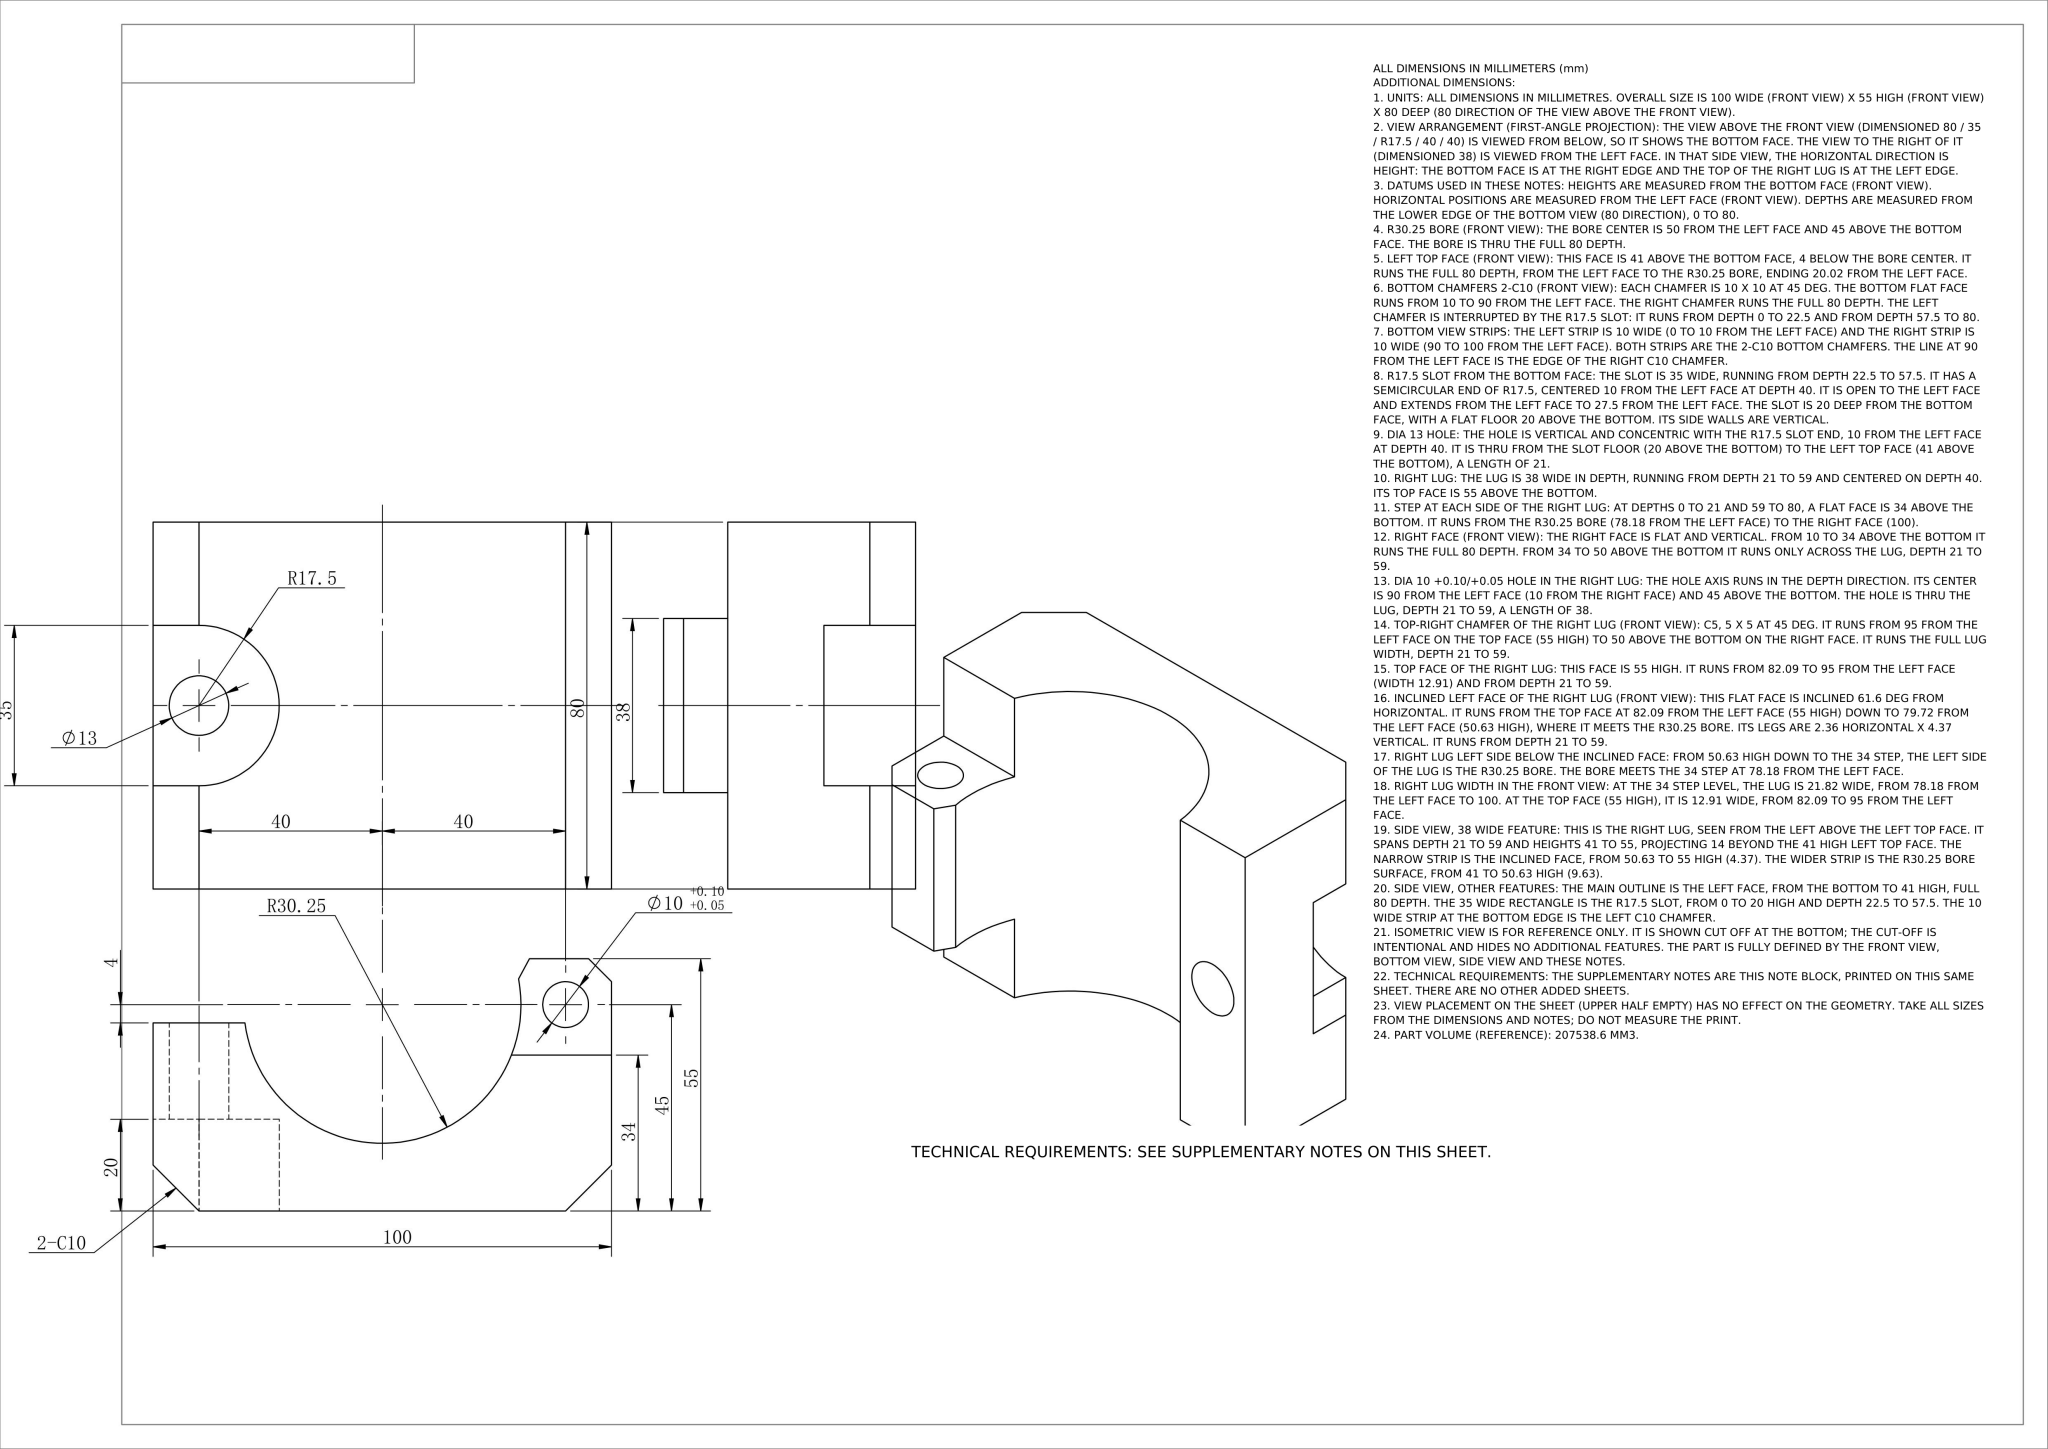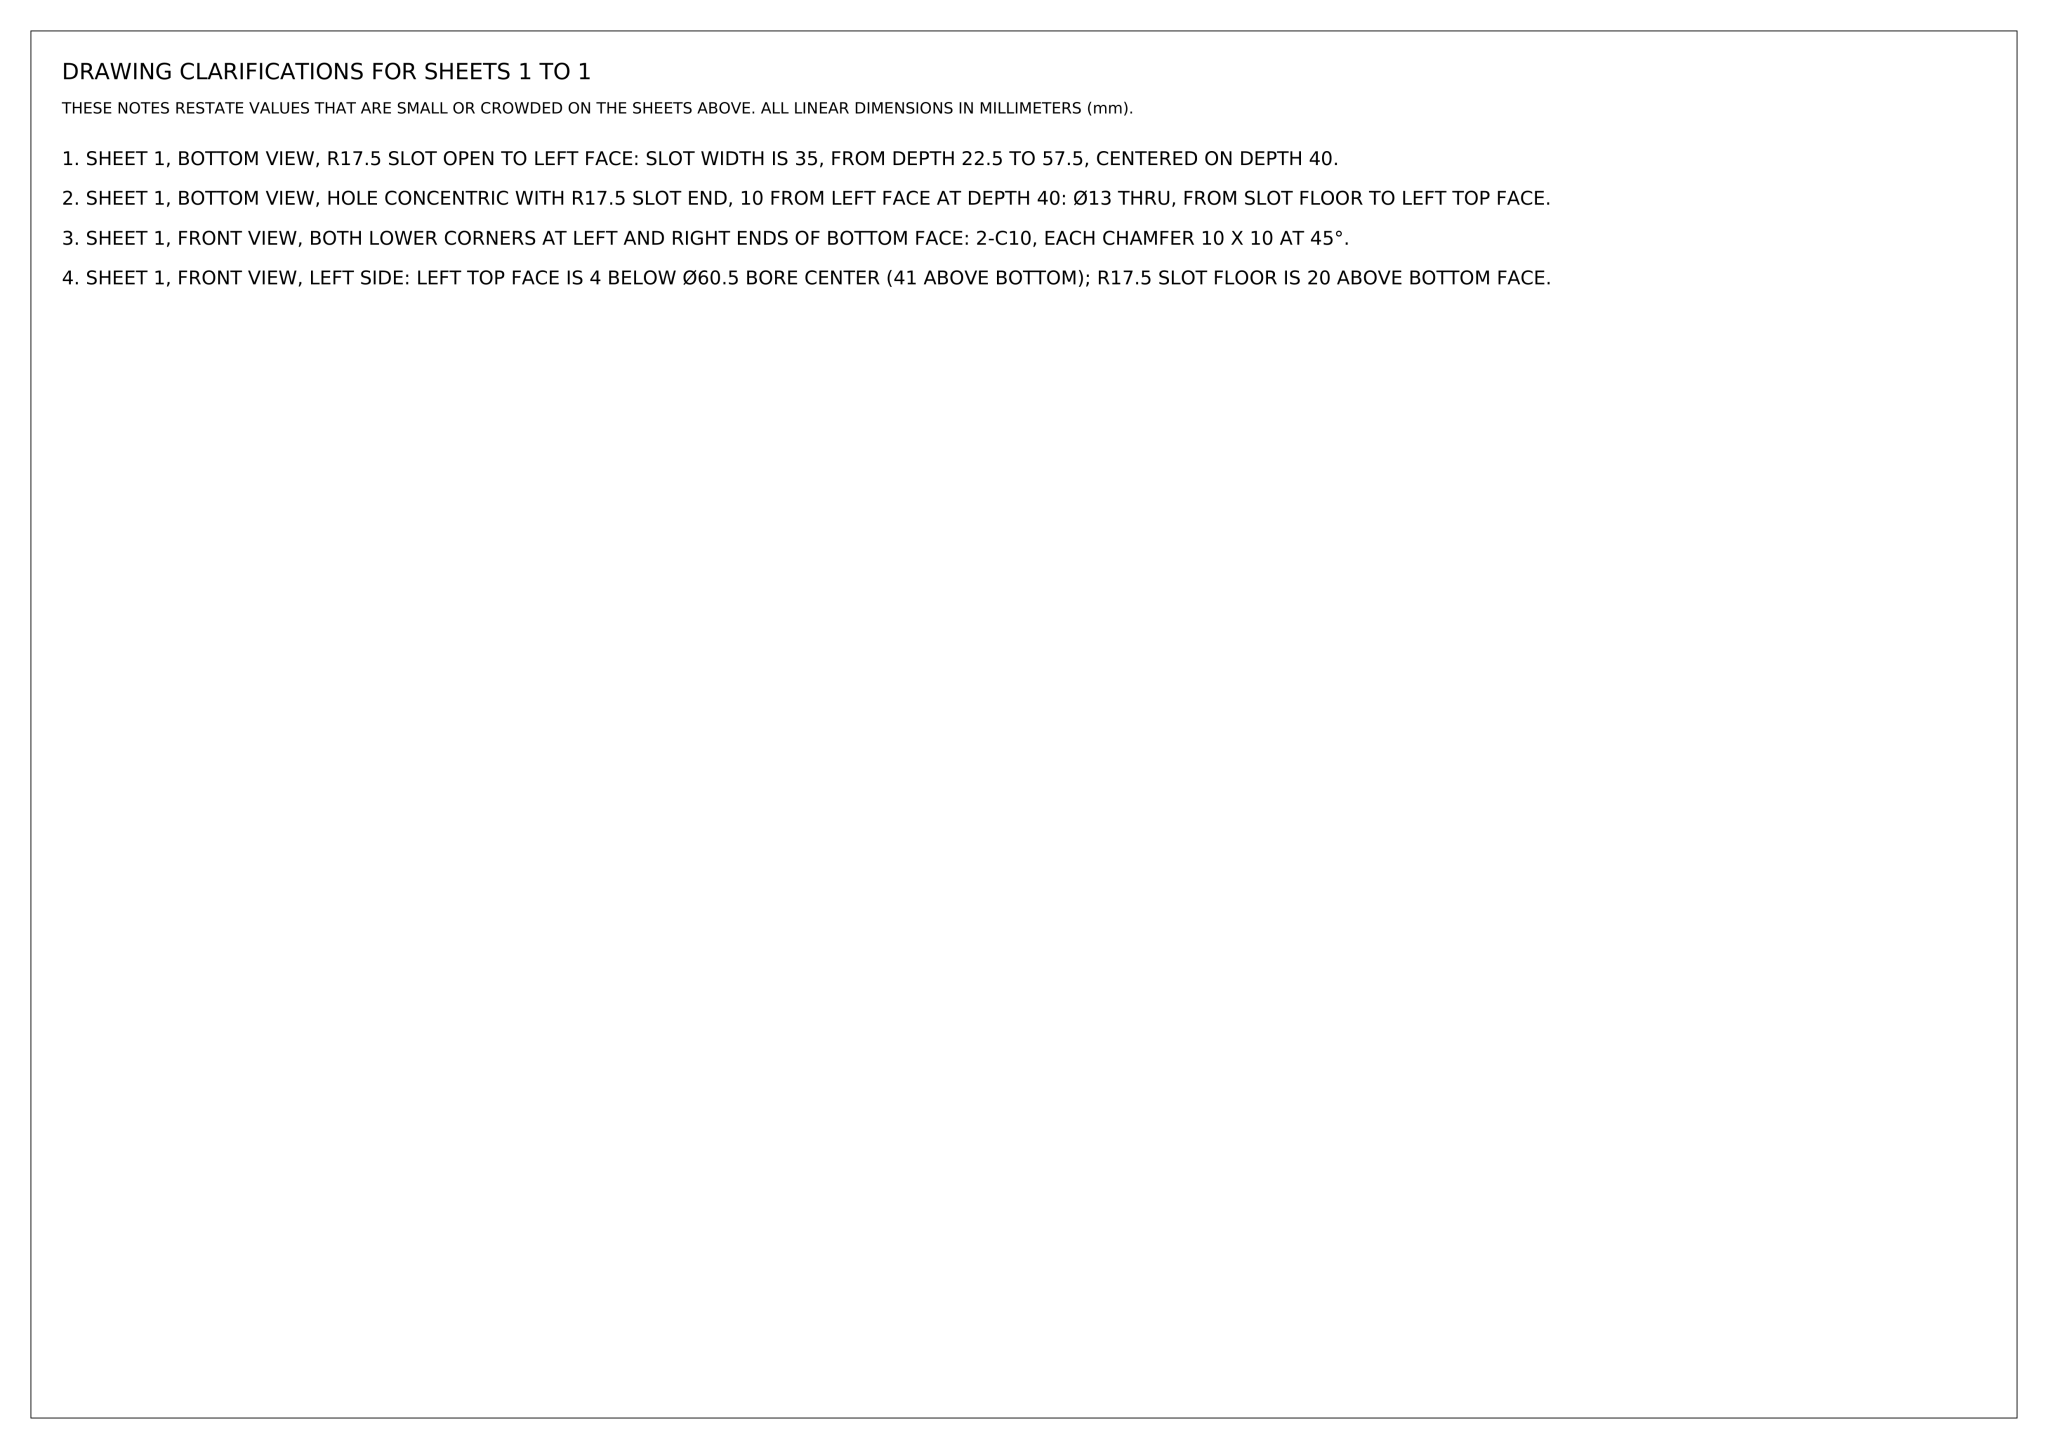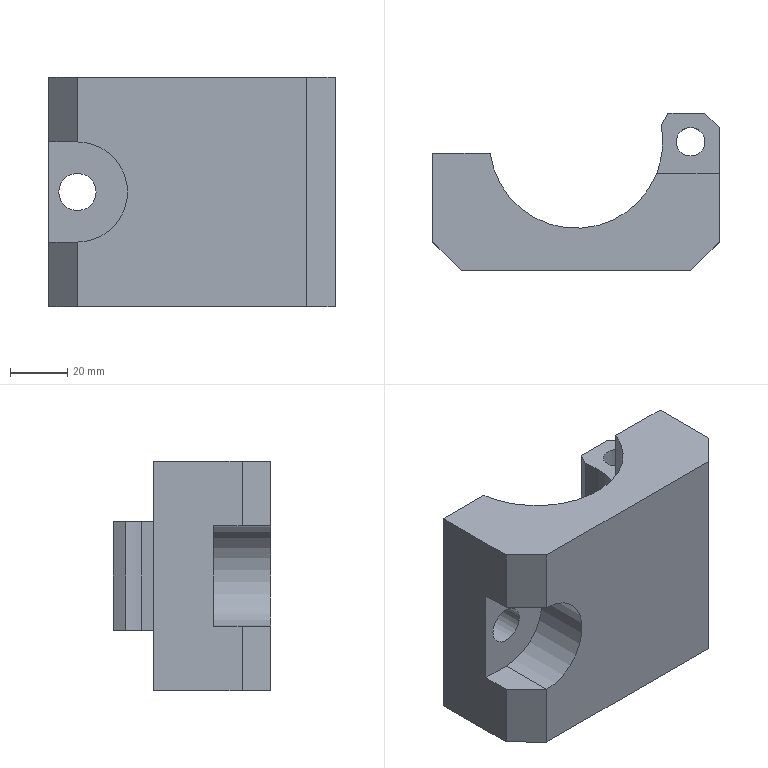Part | NX | mm | 1 solid | 26 faces | box 100 x 55 x 80 mm | volume 207539 mm3 | plane 19 | cylinder 7 | commonest cylinder face diameters 10 x2 60.5 x2 13 x2 35 x1
STEP:
#1=COLOUR_RGB('',0.502,0.502,1.);
#2=FILL_AREA_STYLE_COLOUR('',#1);
#3=FILL_AREA_STYLE('',(#2));
#4=SURFACE_STYLE_FILL_AREA(#3);
#5=SURFACE_SIDE_STYLE('',(#4));
#6=SURFACE_STYLE_USAGE(.BOTH.,#5);
#7=PRESENTATION_STYLE_ASSIGNMENT((#6));
#8=CARTESIAN_POINT('',(45.,-0.,21.));
#9=VERTEX_POINT('',#8);
#10=CARTESIAN_POINT('',(35.,-0.,21.));
#11=VERTEX_POINT('',#10);
#12=CARTESIAN_POINT('',(40.,-0.,21.));
#13=DIRECTION('',(0.,0.,-1.));
#14=DIRECTION('',(0.,-1.,0.));
#15=AXIS2_PLACEMENT_3D('',#12,#13,#14);
#16=CIRCLE('',#15,5.);
#17=EDGE_CURVE('',#9,#11,#16,.T.);
#18=ORIENTED_EDGE('',*,*,#17,.T.);
#19=CARTESIAN_POINT('',(35.,-0.,59.));
#20=VERTEX_POINT('',#19);
#21=CARTESIAN_POINT('',(35.,-0.,-199.));
#22=DIRECTION('',(-0.,-0.,1.));
#23=VECTOR('',#22,1000.);
#24=LINE('',#21,#23);
#25=EDGE_CURVE('',#11,#20,#24,.T.);
#26=ORIENTED_EDGE('',*,*,#25,.T.);
#27=CARTESIAN_POINT('',(45.,-0.,59.));
#28=VERTEX_POINT('',#27);
#29=CARTESIAN_POINT('',(40.,-0.,59.));
#30=DIRECTION('',(-0.,-0.,1.));
#31=DIRECTION('',(-1.,0.,0.));
#32=AXIS2_PLACEMENT_3D('',#29,#30,#31);
#33=CIRCLE('',#32,5.);
#34=EDGE_CURVE('',#20,#28,#33,.T.);
#35=ORIENTED_EDGE('',*,*,#34,.T.);
#36=CARTESIAN_POINT('',(45.,-0.,-199.));
#37=DIRECTION('',(-0.,-0.,1.));
#38=VECTOR('',#37,1000.);
#39=LINE('',#36,#38);
#40=EDGE_CURVE('',#9,#28,#39,.T.);
#41=ORIENTED_EDGE('',*,*,#40,.F.);
#42=EDGE_LOOP('',(#18,#26,#35,#41));
#43=FACE_OUTER_BOUND('',#42,.T.);
#44=CARTESIAN_POINT('',(40.,-0.,-199.));
#45=DIRECTION('',(-0.,-0.,1.));
#46=DIRECTION('',(1.,-0.,0.));
#47=AXIS2_PLACEMENT_3D('',#44,#45,#46);
#48=CYLINDRICAL_SURFACE('',#47,5.);
#49=ADVANCED_FACE('',(#43),#48,.F.);
#50=CARTESIAN_POINT('',(29.722,5.629,21.));
#51=VERTEX_POINT('',#50);
#52=CARTESIAN_POINT('',(30.25,-0.,21.));
#53=VERTEX_POINT('',#52);
#54=CARTESIAN_POINT('',(-0.,-0.,21.));
#55=DIRECTION('',(0.,0.,-1.));
#56=DIRECTION('',(-0.,-1.,-0.));
#57=AXIS2_PLACEMENT_3D('',#54,#55,#56);
#58=CIRCLE('',#57,30.25);
#59=EDGE_CURVE('',#51,#53,#58,.T.);
#60=ORIENTED_EDGE('',*,*,#59,.T.);
#61=CARTESIAN_POINT('',(30.25,-0.,59.));
#62=VERTEX_POINT('',#61);
#63=CARTESIAN_POINT('',(30.25,-0.,-199.));
#64=DIRECTION('',(-0.,-0.,1.));
#65=VECTOR('',#64,1000.);
#66=LINE('',#63,#65);
#67=EDGE_CURVE('',#53,#62,#66,.T.);
#68=ORIENTED_EDGE('',*,*,#67,.T.);
#69=CARTESIAN_POINT('',(29.722,5.629,59.));
#70=VERTEX_POINT('',#69);
#71=CARTESIAN_POINT('',(-0.,-0.,59.));
#72=DIRECTION('',(-0.,-0.,1.));
#73=DIRECTION('',(-1.,0.,0.));
#74=AXIS2_PLACEMENT_3D('',#71,#72,#73);
#75=CIRCLE('',#74,30.25);
#76=EDGE_CURVE('',#62,#70,#75,.T.);
#77=ORIENTED_EDGE('',*,*,#76,.T.);
#78=CARTESIAN_POINT('',(29.722,5.629,-199.));
#79=DIRECTION('',(0.,0.,-1.));
#80=VECTOR('',#79,1000.);
#81=LINE('',#78,#80);
#82=EDGE_CURVE('',#70,#51,#81,.T.);
#83=ORIENTED_EDGE('',*,*,#82,.T.);
#84=EDGE_LOOP('',(#60,#68,#77,#83));
#85=FACE_OUTER_BOUND('',#84,.T.);
#86=CARTESIAN_POINT('',(0.,0.,-199.));
#87=DIRECTION('',(-0.,-0.,1.));
#88=DIRECTION('',(1.,-0.,0.));
#89=AXIS2_PLACEMENT_3D('',#86,#87,#88);
#90=CYLINDRICAL_SURFACE('',#89,30.25);
#91=ADVANCED_FACE('',(#85),#90,.F.);
#92=CARTESIAN_POINT('',(-33.5,-25.,40.));
#93=VERTEX_POINT('',#92);
#94=CARTESIAN_POINT('',(-46.5,-25.,40.));
#95=VERTEX_POINT('',#94);
#96=CARTESIAN_POINT('',(-40.,-25.,40.));
#97=DIRECTION('',(-0.,1.,-0.));
#98=DIRECTION('',(0.,0.,-1.));
#99=AXIS2_PLACEMENT_3D('',#96,#97,#98);
#100=CIRCLE('',#99,6.5);
#101=EDGE_CURVE('',#93,#95,#100,.T.);
#102=ORIENTED_EDGE('',*,*,#101,.F.);
#103=CARTESIAN_POINT('',(-33.5,-4.,40.));
#104=VERTEX_POINT('',#103);
#105=CARTESIAN_POINT('',(-33.5,-75.,40.));
#106=DIRECTION('',(-0.,1.,-0.));
#107=VECTOR('',#106,1000.);
#108=LINE('',#105,#107);
#109=EDGE_CURVE('',#93,#104,#108,.T.);
#110=ORIENTED_EDGE('',*,*,#109,.T.);
#111=CARTESIAN_POINT('',(-46.5,-4.,40.));
#112=VERTEX_POINT('',#111);
#113=CARTESIAN_POINT('',(-40.,-4.,40.));
#114=DIRECTION('',(-0.,1.,-0.));
#115=DIRECTION('',(-1.,0.,0.));
#116=AXIS2_PLACEMENT_3D('',#113,#114,#115);
#117=CIRCLE('',#116,6.5);
#118=EDGE_CURVE('',#104,#112,#117,.T.);
#119=ORIENTED_EDGE('',*,*,#118,.T.);
#120=CARTESIAN_POINT('',(-46.5,-75.,40.));
#121=DIRECTION('',(-0.,1.,-0.));
#122=VECTOR('',#121,1000.);
#123=LINE('',#120,#122);
#124=EDGE_CURVE('',#95,#112,#123,.T.);
#125=ORIENTED_EDGE('',*,*,#124,.F.);
#126=EDGE_LOOP('',(#102,#110,#119,#125));
#127=FACE_OUTER_BOUND('',#126,.T.);
#128=CARTESIAN_POINT('',(-40.,-75.,40.));
#129=DIRECTION('',(-0.,1.,-0.));
#130=DIRECTION('',(-1.,0.,0.));
#131=AXIS2_PLACEMENT_3D('',#128,#129,#130);
#132=CYLINDRICAL_SURFACE('',#131,6.5);
#133=ADVANCED_FACE('',(#127),#132,.F.);
#134=CARTESIAN_POINT('',(-50.,-35.,57.5));
#135=VERTEX_POINT('',#134);
#136=CARTESIAN_POINT('',(-50.,-35.,80.));
#137=VERTEX_POINT('',#136);
#138=CARTESIAN_POINT('',(-50.,-35.,80.));
#139=DIRECTION('',(-0.,-0.,1.));
#140=VECTOR('',#139,1000.);
#141=LINE('',#138,#140);
#142=EDGE_CURVE('',#135,#137,#141,.T.);
#143=ORIENTED_EDGE('',*,*,#142,.F.);
#144=CARTESIAN_POINT('',(-40.,-45.,57.5));
#145=VERTEX_POINT('',#144);
#146=CARTESIAN_POINT('',(-40.,-45.,57.5));
#147=DIRECTION('',(0.7071,-0.7071,0.));
#148=VECTOR('',#147,1000.);
#149=LINE('',#146,#148);
#150=EDGE_CURVE('',#135,#145,#149,.T.);
#151=ORIENTED_EDGE('',*,*,#150,.T.);
#152=CARTESIAN_POINT('',(-40.,-45.,80.));
#153=VERTEX_POINT('',#152);
#154=CARTESIAN_POINT('',(-40.,-45.,80.));
#155=DIRECTION('',(0.,0.,-1.));
#156=VECTOR('',#155,1000.);
#157=LINE('',#154,#156);
#158=EDGE_CURVE('',#153,#145,#157,.T.);
#159=ORIENTED_EDGE('',*,*,#158,.F.);
#160=CARTESIAN_POINT('',(5.,-90.,80.));
#161=DIRECTION('',(0.7071,-0.7071,0.));
#162=VECTOR('',#161,1000.);
#163=LINE('',#160,#162);
#164=EDGE_CURVE('',#137,#153,#163,.T.);
#165=ORIENTED_EDGE('',*,*,#164,.F.);
#166=EDGE_LOOP('',(#143,#151,#159,#165));
#167=FACE_OUTER_BOUND('',#166,.T.);
#168=CARTESIAN_POINT('',(-40.,-45.,80.));
#169=DIRECTION('',(0.7071,0.7071,-0.));
#170=DIRECTION('',(-0.7071,0.7071,-0.));
#171=AXIS2_PLACEMENT_3D('',#168,#169,#170);
#172=PLANE('',#171);
#173=ADVANCED_FACE('',(#167),#172,.F.);
#174=CARTESIAN_POINT('',(-50.,-25.,57.5));
#175=VERTEX_POINT('',#174);
#176=CARTESIAN_POINT('',(-50.,45.,57.5));
#177=DIRECTION('',(-0.,1.,-0.));
#178=VECTOR('',#177,1000.);
#179=LINE('',#176,#178);
#180=EDGE_CURVE('',#135,#175,#179,.T.);
#181=ORIENTED_EDGE('',*,*,#180,.F.);
#182=ORIENTED_EDGE('',*,*,#142,.T.);
#183=CARTESIAN_POINT('',(-50.,-4.,80.));
#184=VERTEX_POINT('',#183);
#185=CARTESIAN_POINT('',(-50.,45.,80.));
#186=DIRECTION('',(0.,-1.,0.));
#187=VECTOR('',#186,1000.);
#188=LINE('',#185,#187);
#189=EDGE_CURVE('',#184,#137,#188,.T.);
#190=ORIENTED_EDGE('',*,*,#189,.F.);
#191=CARTESIAN_POINT('',(-50.,-4.,0.));
#192=VERTEX_POINT('',#191);
#193=CARTESIAN_POINT('',(-50.,-4.,-199.));
#194=DIRECTION('',(-0.,-0.,1.));
#195=VECTOR('',#194,1000.);
#196=LINE('',#193,#195);
#197=EDGE_CURVE('',#192,#184,#196,.T.);
#198=ORIENTED_EDGE('',*,*,#197,.F.);
#199=CARTESIAN_POINT('',(-50.,-35.,0.));
#200=VERTEX_POINT('',#199);
#201=CARTESIAN_POINT('',(-50.,45.,0.));
#202=DIRECTION('',(0.,-1.,0.));
#203=VECTOR('',#202,1000.);
#204=LINE('',#201,#203);
#205=EDGE_CURVE('',#192,#200,#204,.T.);
#206=ORIENTED_EDGE('',*,*,#205,.T.);
#207=CARTESIAN_POINT('',(-50.,-35.,22.5));
#208=VERTEX_POINT('',#207);
#209=CARTESIAN_POINT('',(-50.,-35.,80.));
#210=DIRECTION('',(-0.,-0.,1.));
#211=VECTOR('',#210,1000.);
#212=LINE('',#209,#211);
#213=EDGE_CURVE('',#200,#208,#212,.T.);
#214=ORIENTED_EDGE('',*,*,#213,.T.);
#215=CARTESIAN_POINT('',(-50.,-25.,22.5));
#216=VERTEX_POINT('',#215);
#217=CARTESIAN_POINT('',(-50.,45.,22.5));
#218=DIRECTION('',(0.,-1.,0.));
#219=VECTOR('',#218,1000.);
#220=LINE('',#217,#219);
#221=EDGE_CURVE('',#216,#208,#220,.T.);
#222=ORIENTED_EDGE('',*,*,#221,.F.);
#223=CARTESIAN_POINT('',(-50.,-25.,80.));
#224=DIRECTION('',(0.,0.,-1.));
#225=VECTOR('',#224,1000.);
#226=LINE('',#223,#225);
#227=EDGE_CURVE('',#175,#216,#226,.T.);
#228=ORIENTED_EDGE('',*,*,#227,.F.);
#229=EDGE_LOOP('',(#181,#182,#190,#198,#206,#214,#222,#228));
#230=FACE_OUTER_BOUND('',#229,.T.);
#231=CARTESIAN_POINT('',(-50.,45.,80.));
#232=DIRECTION('',(1.,0.,-0.));
#233=DIRECTION('',(-0.,1.,-0.));
#234=AXIS2_PLACEMENT_3D('',#231,#232,#233);
#235=PLANE('',#234);
#236=ADVANCED_FACE('',(#230),#235,.F.);
#237=CARTESIAN_POINT('',(-40.,-45.,22.5));
#238=VERTEX_POINT('',#237);
#239=CARTESIAN_POINT('',(-40.,-45.,0.));
#240=VERTEX_POINT('',#239);
#241=CARTESIAN_POINT('',(-40.,-45.,80.));
#242=DIRECTION('',(0.,0.,-1.));
#243=VECTOR('',#242,1000.);
#244=LINE('',#241,#243);
#245=EDGE_CURVE('',#238,#240,#244,.T.);
#246=ORIENTED_EDGE('',*,*,#245,.F.);
#247=CARTESIAN_POINT('',(-40.,-45.,22.5));
#248=DIRECTION('',(-0.7071,0.7071,0.));
#249=VECTOR('',#248,1000.);
#250=LINE('',#247,#249);
#251=EDGE_CURVE('',#238,#208,#250,.T.);
#252=ORIENTED_EDGE('',*,*,#251,.T.);
#253=ORIENTED_EDGE('',*,*,#213,.F.);
#254=CARTESIAN_POINT('',(-40.,-45.,0.));
#255=DIRECTION('',(-0.7071,0.7071,-0.));
#256=VECTOR('',#255,1000.);
#257=LINE('',#254,#256);
#258=EDGE_CURVE('',#240,#200,#257,.T.);
#259=ORIENTED_EDGE('',*,*,#258,.F.);
#260=EDGE_LOOP('',(#246,#252,#253,#259));
#261=FACE_OUTER_BOUND('',#260,.T.);
#262=CARTESIAN_POINT('',(-40.,-45.,80.));
#263=DIRECTION('',(0.7071,0.7071,-0.));
#264=DIRECTION('',(-0.7071,0.7071,-0.));
#265=AXIS2_PLACEMENT_3D('',#262,#263,#264);
#266=PLANE('',#265);
#267=ADVANCED_FACE('',(#261),#266,.F.);
#268=CARTESIAN_POINT('',(-40.,-45.,40.));
#269=DIRECTION('',(0.,-1.,0.));
#270=DIRECTION('',(0.,0.,-1.));
#271=AXIS2_PLACEMENT_3D('',#268,#269,#270);
#272=CIRCLE('',#271,17.5);
#273=EDGE_CURVE('',#238,#145,#272,.T.);
#274=ORIENTED_EDGE('',*,*,#273,.T.);
#275=CARTESIAN_POINT('',(-40.,-25.,57.5));
#276=VERTEX_POINT('',#275);
#277=CARTESIAN_POINT('',(-40.,-65.,57.5));
#278=DIRECTION('',(-0.,1.,-0.));
#279=VECTOR('',#278,1000.);
#280=LINE('',#277,#279);
#281=EDGE_CURVE('',#145,#276,#280,.T.);
#282=ORIENTED_EDGE('',*,*,#281,.T.);
#283=CARTESIAN_POINT('',(-40.,-25.,22.5));
#284=VERTEX_POINT('',#283);
#285=CARTESIAN_POINT('',(-40.,-25.,40.));
#286=DIRECTION('',(0.,-1.,0.));
#287=DIRECTION('',(0.,0.,-1.));
#288=AXIS2_PLACEMENT_3D('',#285,#286,#287);
#289=CIRCLE('',#288,17.5);
#290=EDGE_CURVE('',#284,#276,#289,.T.);
#291=ORIENTED_EDGE('',*,*,#290,.F.);
#292=CARTESIAN_POINT('',(-40.,-65.,22.5));
#293=DIRECTION('',(-0.,1.,-0.));
#294=VECTOR('',#293,1000.);
#295=LINE('',#292,#294);
#296=EDGE_CURVE('',#238,#284,#295,.T.);
#297=ORIENTED_EDGE('',*,*,#296,.F.);
#298=EDGE_LOOP('',(#274,#282,#291,#297));
#299=FACE_OUTER_BOUND('',#298,.T.);
#300=CARTESIAN_POINT('',(-40.,-25.,40.));
#301=DIRECTION('',(0.,-1.,0.));
#302=DIRECTION('',(0.,0.,-1.));
#303=AXIS2_PLACEMENT_3D('',#300,#301,#302);
#304=CYLINDRICAL_SURFACE('',#303,17.5);
#305=ADVANCED_FACE('',(#299),#304,.F.);
#306=ORIENTED_EDGE('',*,*,#109,.F.);
#307=CARTESIAN_POINT('',(-40.,-25.,40.));
#308=DIRECTION('',(-0.,1.,-0.));
#309=DIRECTION('',(0.,0.,-1.));
#310=AXIS2_PLACEMENT_3D('',#307,#308,#309);
#311=CIRCLE('',#310,6.5);
#312=EDGE_CURVE('',#95,#93,#311,.T.);
#313=ORIENTED_EDGE('',*,*,#312,.F.);
#314=ORIENTED_EDGE('',*,*,#124,.T.);
#315=CARTESIAN_POINT('',(-40.,-4.,40.));
#316=DIRECTION('',(-0.,1.,-0.));
#317=DIRECTION('',(-1.,0.,0.));
#318=AXIS2_PLACEMENT_3D('',#315,#316,#317);
#319=CIRCLE('',#318,6.5);
#320=EDGE_CURVE('',#112,#104,#319,.T.);
#321=ORIENTED_EDGE('',*,*,#320,.T.);
#322=EDGE_LOOP('',(#306,#313,#314,#321));
#323=FACE_OUTER_BOUND('',#322,.T.);
#324=CARTESIAN_POINT('',(-40.,-75.,40.));
#325=DIRECTION('',(-0.,1.,-0.));
#326=DIRECTION('',(-1.,0.,0.));
#327=AXIS2_PLACEMENT_3D('',#324,#325,#326);
#328=CYLINDRICAL_SURFACE('',#327,6.5);
#329=ADVANCED_FACE('',(#323),#328,.F.);
#330=CARTESIAN_POINT('',(50.,-35.,80.));
#331=VERTEX_POINT('',#330);
#332=CARTESIAN_POINT('',(50.,-11.,80.));
#333=VERTEX_POINT('',#332);
#334=CARTESIAN_POINT('',(50.,45.,80.));
#335=DIRECTION('',(-0.,1.,-0.));
#336=VECTOR('',#335,1000.);
#337=LINE('',#334,#336);
#338=EDGE_CURVE('',#331,#333,#337,.T.);
#339=ORIENTED_EDGE('',*,*,#338,.F.);
#340=CARTESIAN_POINT('',(50.,-35.,0.));
#341=VERTEX_POINT('',#340);
#342=CARTESIAN_POINT('',(50.,-35.,80.));
#343=DIRECTION('',(0.,0.,-1.));
#344=VECTOR('',#343,1000.);
#345=LINE('',#342,#344);
#346=EDGE_CURVE('',#331,#341,#345,.T.);
#347=ORIENTED_EDGE('',*,*,#346,.T.);
#348=CARTESIAN_POINT('',(50.,-11.,0.));
#349=VERTEX_POINT('',#348);
#350=CARTESIAN_POINT('',(50.,45.,0.));
#351=DIRECTION('',(-0.,1.,-0.));
#352=VECTOR('',#351,1000.);
#353=LINE('',#350,#352);
#354=EDGE_CURVE('',#341,#349,#353,.T.);
#355=ORIENTED_EDGE('',*,*,#354,.T.);
#356=CARTESIAN_POINT('',(50.,-11.,21.));
#357=VERTEX_POINT('',#356);
#358=CARTESIAN_POINT('',(50.,-11.,0.));
#359=DIRECTION('',(0.,0.,-1.));
#360=VECTOR('',#359,1000.);
#361=LINE('',#358,#360);
#362=EDGE_CURVE('',#357,#349,#361,.T.);
#363=ORIENTED_EDGE('',*,*,#362,.F.);
#364=CARTESIAN_POINT('',(50.,5.,21.));
#365=VERTEX_POINT('',#364);
#366=CARTESIAN_POINT('',(50.,10.,21.));
#367=DIRECTION('',(0.,-1.,-0.));
#368=VECTOR('',#367,1000.);
#369=LINE('',#366,#368);
#370=EDGE_CURVE('',#365,#357,#369,.T.);
#371=ORIENTED_EDGE('',*,*,#370,.F.);
#372=CARTESIAN_POINT('',(50.,5.,59.));
#373=VERTEX_POINT('',#372);
#374=CARTESIAN_POINT('',(50.,5.,80.));
#375=DIRECTION('',(-0.,-0.,1.));
#376=VECTOR('',#375,1000.);
#377=LINE('',#374,#376);
#378=EDGE_CURVE('',#365,#373,#377,.T.);
#379=ORIENTED_EDGE('',*,*,#378,.T.);
#380=CARTESIAN_POINT('',(50.,-11.,59.));
#381=VERTEX_POINT('',#380);
#382=CARTESIAN_POINT('',(50.,10.,59.));
#383=DIRECTION('',(-0.,1.,-0.));
#384=VECTOR('',#383,1000.);
#385=LINE('',#382,#384);
#386=EDGE_CURVE('',#381,#373,#385,.T.);
#387=ORIENTED_EDGE('',*,*,#386,.F.);
#388=CARTESIAN_POINT('',(50.,-11.,80.));
#389=DIRECTION('',(0.,0.,-1.));
#390=VECTOR('',#389,1000.);
#391=LINE('',#388,#390);
#392=EDGE_CURVE('',#333,#381,#391,.T.);
#393=ORIENTED_EDGE('',*,*,#392,.F.);
#394=EDGE_LOOP('',(#339,#347,#355,#363,#371,#379,#387,#393));
#395=FACE_OUTER_BOUND('',#394,.T.);
#396=CARTESIAN_POINT('',(50.,45.,80.));
#397=DIRECTION('',(-1.,-0.,0.));
#398=DIRECTION('',(0.,-1.,0.));
#399=AXIS2_PLACEMENT_3D('',#396,#397,#398);
#400=PLANE('',#399);
#401=ADVANCED_FACE('',(#395),#400,.F.);
#402=ORIENTED_EDGE('',*,*,#158,.T.);
#403=ORIENTED_EDGE('',*,*,#273,.F.);
#404=ORIENTED_EDGE('',*,*,#245,.T.);
#405=CARTESIAN_POINT('',(40.,-45.,0.));
#406=VERTEX_POINT('',#405);
#407=CARTESIAN_POINT('',(-50.,-45.,0.));
#408=DIRECTION('',(1.,-0.,-0.));
#409=VECTOR('',#408,1000.);
#410=LINE('',#407,#409);
#411=EDGE_CURVE('',#240,#406,#410,.T.);
#412=ORIENTED_EDGE('',*,*,#411,.T.);
#413=CARTESIAN_POINT('',(40.,-45.,80.));
#414=VERTEX_POINT('',#413);
#415=CARTESIAN_POINT('',(40.,-45.,80.));
#416=DIRECTION('',(-0.,-0.,1.));
#417=VECTOR('',#416,1000.);
#418=LINE('',#415,#417);
#419=EDGE_CURVE('',#406,#414,#418,.T.);
#420=ORIENTED_EDGE('',*,*,#419,.T.);
#421=CARTESIAN_POINT('',(-50.,-45.,80.));
#422=DIRECTION('',(1.,-0.,-0.));
#423=VECTOR('',#422,1000.);
#424=LINE('',#421,#423);
#425=EDGE_CURVE('',#153,#414,#424,.T.);
#426=ORIENTED_EDGE('',*,*,#425,.F.);
#427=EDGE_LOOP('',(#402,#403,#404,#412,#420,#426));
#428=FACE_OUTER_BOUND('',#427,.T.);
#429=CARTESIAN_POINT('',(-50.,-45.,80.));
#430=DIRECTION('',(-0.,1.,0.));
#431=DIRECTION('',(-0.,-0.,1.));
#432=AXIS2_PLACEMENT_3D('',#429,#430,#431);
#433=PLANE('',#432);
#434=ADVANCED_FACE('',(#428),#433,.F.);
#435=ORIENTED_EDGE('',*,*,#189,.T.);
#436=ORIENTED_EDGE('',*,*,#164,.T.);
#437=ORIENTED_EDGE('',*,*,#425,.T.);
#438=CARTESIAN_POINT('',(45.,-40.,80.));
#439=DIRECTION('',(0.7071,0.7071,-0.));
#440=VECTOR('',#439,1000.);
#441=LINE('',#438,#440);
#442=EDGE_CURVE('',#414,#331,#441,.T.);
#443=ORIENTED_EDGE('',*,*,#442,.T.);
#444=ORIENTED_EDGE('',*,*,#338,.T.);
#445=CARTESIAN_POINT('',(28.179,-11.,80.));
#446=VERTEX_POINT('',#445);
#447=CARTESIAN_POINT('',(-9.,-11.,80.));
#448=DIRECTION('',(1.,-0.,-0.));
#449=VECTOR('',#448,1000.);
#450=LINE('',#447,#449);
#451=EDGE_CURVE('',#446,#333,#450,.T.);
#452=ORIENTED_EDGE('',*,*,#451,.F.);
#453=CARTESIAN_POINT('',(-29.984,-4.,80.));
#454=VERTEX_POINT('',#453);
#455=CARTESIAN_POINT('',(-0.,-0.,80.));
#456=DIRECTION('',(-0.,-0.,1.));
#457=DIRECTION('',(1.,-0.,0.));
#458=AXIS2_PLACEMENT_3D('',#455,#456,#457);
#459=CIRCLE('',#458,30.25);
#460=EDGE_CURVE('',#454,#446,#459,.T.);
#461=ORIENTED_EDGE('',*,*,#460,.F.);
#462=CARTESIAN_POINT('',(0.,-4.,80.));
#463=DIRECTION('',(1.,-0.,-0.));
#464=VECTOR('',#463,1000.);
#465=LINE('',#462,#464);
#466=EDGE_CURVE('',#184,#454,#465,.T.);
#467=ORIENTED_EDGE('',*,*,#466,.F.);
#468=EDGE_LOOP('',(#435,#436,#437,#443,#444,#452,#461,#467));
#469=FACE_OUTER_BOUND('',#468,.T.);
#470=CARTESIAN_POINT('',(50.,-45.,80.));
#471=DIRECTION('',(0.,-0.,1.));
#472=DIRECTION('',(1.,-0.,-0.));
#473=AXIS2_PLACEMENT_3D('',#470,#471,#472);
#474=PLANE('',#473);
#475=ADVANCED_FACE('',(#469),#474,.T.);
#476=ORIENTED_EDGE('',*,*,#411,.F.);
#477=ORIENTED_EDGE('',*,*,#258,.T.);
#478=ORIENTED_EDGE('',*,*,#205,.F.);
#479=CARTESIAN_POINT('',(-29.984,-4.,0.));
#480=VERTEX_POINT('',#479);
#481=CARTESIAN_POINT('',(50.,-4.,0.));
#482=DIRECTION('',(1.,-0.,-0.));
#483=VECTOR('',#482,1000.);
#484=LINE('',#481,#483);
#485=EDGE_CURVE('',#192,#480,#484,.T.);
#486=ORIENTED_EDGE('',*,*,#485,.T.);
#487=CARTESIAN_POINT('',(28.179,-11.,0.));
#488=VERTEX_POINT('',#487);
#489=CARTESIAN_POINT('',(0.,0.,0.));
#490=DIRECTION('',(-0.,-0.,1.));
#491=DIRECTION('',(1.,-0.,-0.));
#492=AXIS2_PLACEMENT_3D('',#489,#490,#491);
#493=CIRCLE('',#492,30.25);
#494=EDGE_CURVE('',#480,#488,#493,.T.);
#495=ORIENTED_EDGE('',*,*,#494,.T.);
#496=CARTESIAN_POINT('',(-9.,-11.,0.));
#497=DIRECTION('',(1.,-0.,-0.));
#498=VECTOR('',#497,1000.);
#499=LINE('',#496,#498);
#500=EDGE_CURVE('',#488,#349,#499,.T.);
#501=ORIENTED_EDGE('',*,*,#500,.T.);
#502=ORIENTED_EDGE('',*,*,#354,.F.);
#503=CARTESIAN_POINT('',(50.,-35.,0.));
#504=DIRECTION('',(-0.7071,-0.7071,0.));
#505=VECTOR('',#504,1000.);
#506=LINE('',#503,#505);
#507=EDGE_CURVE('',#341,#406,#506,.T.);
#508=ORIENTED_EDGE('',*,*,#507,.T.);
#509=EDGE_LOOP('',(#476,#477,#478,#486,#495,#501,#502,#508));
#510=FACE_OUTER_BOUND('',#509,.T.);
#511=CARTESIAN_POINT('',(50.,-45.,0.));
#512=DIRECTION('',(0.,-0.,1.));
#513=DIRECTION('',(1.,-0.,-0.));
#514=AXIS2_PLACEMENT_3D('',#511,#512,#513);
#515=PLANE('',#514);
#516=ADVANCED_FACE('',(#510),#515,.F.);
#517=ORIENTED_EDGE('',*,*,#67,.F.);
#518=CARTESIAN_POINT('',(28.179,-11.,21.));
#519=VERTEX_POINT('',#518);
#520=CARTESIAN_POINT('',(-0.,-0.,21.));
#521=DIRECTION('',(0.,0.,-1.));
#522=DIRECTION('',(0.,-1.,-0.));
#523=AXIS2_PLACEMENT_3D('',#520,#521,#522);
#524=CIRCLE('',#523,30.25);
#525=EDGE_CURVE('',#53,#519,#524,.T.);
#526=ORIENTED_EDGE('',*,*,#525,.T.);
#527=CARTESIAN_POINT('',(28.179,-11.,-199.));
#528=DIRECTION('',(0.,0.,-1.));
#529=VECTOR('',#528,1000.);
#530=LINE('',#527,#529);
#531=EDGE_CURVE('',#519,#488,#530,.T.);
#532=ORIENTED_EDGE('',*,*,#531,.T.);
#533=ORIENTED_EDGE('',*,*,#494,.F.);
#534=CARTESIAN_POINT('',(-29.984,-4.,-199.));
#535=DIRECTION('',(-0.,-0.,1.));
#536=VECTOR('',#535,1000.);
#537=LINE('',#534,#536);
#538=EDGE_CURVE('',#480,#454,#537,.T.);
#539=ORIENTED_EDGE('',*,*,#538,.T.);
#540=ORIENTED_EDGE('',*,*,#460,.T.);
#541=CARTESIAN_POINT('',(28.179,-11.,59.));
#542=VERTEX_POINT('',#541);
#543=CARTESIAN_POINT('',(28.179,-11.,-199.));
#544=DIRECTION('',(0.,0.,-1.));
#545=VECTOR('',#544,1000.);
#546=LINE('',#543,#545);
#547=EDGE_CURVE('',#446,#542,#546,.T.);
#548=ORIENTED_EDGE('',*,*,#547,.T.);
#549=CARTESIAN_POINT('',(-0.,-0.,59.));
#550=DIRECTION('',(-0.,-0.,1.));
#551=DIRECTION('',(-1.,0.,0.));
#552=AXIS2_PLACEMENT_3D('',#549,#550,#551);
#553=CIRCLE('',#552,30.25);
#554=EDGE_CURVE('',#542,#62,#553,.T.);
#555=ORIENTED_EDGE('',*,*,#554,.T.);
#556=EDGE_LOOP('',(#517,#526,#532,#533,#539,#540,#548,#555));
#557=FACE_OUTER_BOUND('',#556,.T.);
#558=CARTESIAN_POINT('',(0.,0.,-199.));
#559=DIRECTION('',(-0.,-0.,1.));
#560=DIRECTION('',(1.,-0.,0.));
#561=AXIS2_PLACEMENT_3D('',#558,#559,#560);
#562=CYLINDRICAL_SURFACE('',#561,30.25);
#563=ADVANCED_FACE('',(#557),#562,.F.);
#564=ORIENTED_EDGE('',*,*,#25,.F.);
#565=CARTESIAN_POINT('',(40.,-0.,21.));
#566=DIRECTION('',(0.,0.,-1.));
#567=DIRECTION('',(0.,-1.,0.));
#568=AXIS2_PLACEMENT_3D('',#565,#566,#567);
#569=CIRCLE('',#568,5.);
#570=EDGE_CURVE('',#11,#9,#569,.T.);
#571=ORIENTED_EDGE('',*,*,#570,.T.);
#572=ORIENTED_EDGE('',*,*,#40,.T.);
#573=CARTESIAN_POINT('',(40.,-0.,59.));
#574=DIRECTION('',(-0.,-0.,1.));
#575=DIRECTION('',(-1.,0.,0.));
#576=AXIS2_PLACEMENT_3D('',#573,#574,#575);
#577=CIRCLE('',#576,5.);
#578=EDGE_CURVE('',#28,#20,#577,.T.);
#579=ORIENTED_EDGE('',*,*,#578,.T.);
#580=EDGE_LOOP('',(#564,#571,#572,#579));
#581=FACE_OUTER_BOUND('',#580,.T.);
#582=CARTESIAN_POINT('',(40.,-0.,-199.));
#583=DIRECTION('',(-0.,-0.,1.));
#584=DIRECTION('',(1.,-0.,0.));
#585=AXIS2_PLACEMENT_3D('',#582,#583,#584);
#586=CYLINDRICAL_SURFACE('',#585,5.);
#587=ADVANCED_FACE('',(#581),#586,.F.);
#588=CARTESIAN_POINT('',(45.,10.,59.));
#589=VERTEX_POINT('',#588);
#590=CARTESIAN_POINT('',(45.,10.,21.));
#591=VERTEX_POINT('',#590);
#592=CARTESIAN_POINT('',(45.,10.,-199.));
#593=DIRECTION('',(0.,0.,-1.));
#594=VECTOR('',#593,1000.);
#595=LINE('',#592,#594);
#596=EDGE_CURVE('',#589,#591,#595,.T.);
#597=ORIENTED_EDGE('',*,*,#596,.T.);
#598=CARTESIAN_POINT('',(32.086,10.,21.));
#599=VERTEX_POINT('',#598);
#600=CARTESIAN_POINT('',(-9.,10.,21.));
#601=DIRECTION('',(1.,-0.,-0.));
#602=VECTOR('',#601,1000.);
#603=LINE('',#600,#602);
#604=EDGE_CURVE('',#599,#591,#603,.T.);
#605=ORIENTED_EDGE('',*,*,#604,.F.);
#606=CARTESIAN_POINT('',(32.086,10.,59.));
#607=VERTEX_POINT('',#606);
#608=CARTESIAN_POINT('',(32.086,10.,-199.));
#609=DIRECTION('',(-0.,-0.,1.));
#610=VECTOR('',#609,1000.);
#611=LINE('',#608,#610);
#612=EDGE_CURVE('',#599,#607,#611,.T.);
#613=ORIENTED_EDGE('',*,*,#612,.T.);
#614=CARTESIAN_POINT('',(-9.,10.,59.));
#615=DIRECTION('',(1.,-0.,-0.));
#616=VECTOR('',#615,1000.);
#617=LINE('',#614,#616);
#618=EDGE_CURVE('',#607,#589,#617,.T.);
#619=ORIENTED_EDGE('',*,*,#618,.T.);
#620=EDGE_LOOP('',(#597,#605,#613,#619));
#621=FACE_OUTER_BOUND('',#620,.T.);
#622=CARTESIAN_POINT('',(50.,10.,-199.));
#623=DIRECTION('',(-0.,-1.,0.));
#624=DIRECTION('',(1.,-0.,-0.));
#625=AXIS2_PLACEMENT_3D('',#622,#623,#624);
#626=PLANE('',#625);
#627=ADVANCED_FACE('',(#621),#626,.F.);
#628=ORIENTED_EDGE('',*,*,#320,.F.);
#629=ORIENTED_EDGE('',*,*,#118,.F.);
#630=EDGE_LOOP('',(#628,#629));
#631=FACE_BOUND('',#630,.T.);
#632=ORIENTED_EDGE('',*,*,#197,.T.);
#633=ORIENTED_EDGE('',*,*,#466,.T.);
#634=ORIENTED_EDGE('',*,*,#538,.F.);
#635=ORIENTED_EDGE('',*,*,#485,.F.);
#636=EDGE_LOOP('',(#632,#633,#634,#635));
#637=FACE_OUTER_BOUND('',#636,.T.);
#638=CARTESIAN_POINT('',(0.,-4.,-199.));
#639=DIRECTION('',(-0.,-1.,0.));
#640=DIRECTION('',(1.,-0.,-0.));
#641=AXIS2_PLACEMENT_3D('',#638,#639,#640);
#642=PLANE('',#641);
#643=ADVANCED_FACE('',(#631,#637),#642,.F.);
#644=CARTESIAN_POINT('',(29.722,5.629,21.));
#645=DIRECTION('',(0.4757,0.8796,0.));
#646=VECTOR('',#645,1000.);
#647=LINE('',#644,#646);
#648=EDGE_CURVE('',#51,#599,#647,.T.);
#649=ORIENTED_EDGE('',*,*,#648,.F.);
#650=ORIENTED_EDGE('',*,*,#82,.F.);
#651=CARTESIAN_POINT('',(29.722,5.629,59.));
#652=DIRECTION('',(-0.4757,-0.8796,0.));
#653=VECTOR('',#652,1000.);
#654=LINE('',#651,#653);
#655=EDGE_CURVE('',#607,#70,#654,.T.);
#656=ORIENTED_EDGE('',*,*,#655,.F.);
#657=ORIENTED_EDGE('',*,*,#612,.F.);
#658=EDGE_LOOP('',(#649,#650,#656,#657));
#659=FACE_OUTER_BOUND('',#658,.T.);
#660=CARTESIAN_POINT('',(29.722,5.629,-199.));
#661=DIRECTION('',(-0.8796,0.4757,0.));
#662=DIRECTION('',(-0.4757,-0.8796,0.));
#663=AXIS2_PLACEMENT_3D('',#660,#661,#662);
#664=PLANE('',#663);
#665=ADVANCED_FACE('',(#659),#664,.T.);
#666=CARTESIAN_POINT('',(50.,5.,21.));
#667=DIRECTION('',(0.7071,-0.7071,-0.));
#668=VECTOR('',#667,1000.);
#669=LINE('',#666,#668);
#670=EDGE_CURVE('',#591,#365,#669,.T.);
#671=ORIENTED_EDGE('',*,*,#670,.F.);
#672=ORIENTED_EDGE('',*,*,#596,.F.);
#673=CARTESIAN_POINT('',(50.,5.,59.));
#674=DIRECTION('',(-0.7071,0.7071,-0.));
#675=VECTOR('',#674,1000.);
#676=LINE('',#673,#675);
#677=EDGE_CURVE('',#373,#589,#676,.T.);
#678=ORIENTED_EDGE('',*,*,#677,.F.);
#679=ORIENTED_EDGE('',*,*,#378,.F.);
#680=EDGE_LOOP('',(#671,#672,#678,#679));
#681=FACE_OUTER_BOUND('',#680,.T.);
#682=CARTESIAN_POINT('',(50.,5.,80.));
#683=DIRECTION('',(-0.7071,-0.7071,0.));
#684=DIRECTION('',(0.7071,-0.7071,0.));
#685=AXIS2_PLACEMENT_3D('',#682,#683,#684);
#686=PLANE('',#685);
#687=ADVANCED_FACE('',(#681),#686,.F.);
#688=ORIENTED_EDGE('',*,*,#451,.T.);
#689=ORIENTED_EDGE('',*,*,#392,.T.);
#690=CARTESIAN_POINT('',(-9.,-11.,59.));
#691=DIRECTION('',(1.,-0.,-0.));
#692=VECTOR('',#691,1000.);
#693=LINE('',#690,#692);
#694=EDGE_CURVE('',#542,#381,#693,.T.);
#695=ORIENTED_EDGE('',*,*,#694,.F.);
#696=ORIENTED_EDGE('',*,*,#547,.F.);
#697=EDGE_LOOP('',(#688,#689,#695,#696));
#698=FACE_OUTER_BOUND('',#697,.T.);
#699=CARTESIAN_POINT('',(-9.,-11.,80.));
#700=DIRECTION('',(-0.,-1.,0.));
#701=DIRECTION('',(1.,-0.,-0.));
#702=AXIS2_PLACEMENT_3D('',#699,#700,#701);
#703=PLANE('',#702);
#704=ADVANCED_FACE('',(#698),#703,.F.);
#705=ORIENTED_EDGE('',*,*,#694,.T.);
#706=ORIENTED_EDGE('',*,*,#386,.T.);
#707=ORIENTED_EDGE('',*,*,#677,.T.);
#708=ORIENTED_EDGE('',*,*,#618,.F.);
#709=ORIENTED_EDGE('',*,*,#655,.T.);
#710=ORIENTED_EDGE('',*,*,#76,.F.);
#711=ORIENTED_EDGE('',*,*,#554,.F.);
#712=EDGE_LOOP('',(#705,#706,#707,#708,#709,#710,#711));
#713=FACE_OUTER_BOUND('',#712,.T.);
#714=ORIENTED_EDGE('',*,*,#578,.F.);
#715=ORIENTED_EDGE('',*,*,#34,.F.);
#716=EDGE_LOOP('',(#714,#715));
#717=FACE_BOUND('',#716,.T.);
#718=CARTESIAN_POINT('',(-9.,10.,59.));
#719=DIRECTION('',(-0.,0.,-1.));
#720=DIRECTION('',(-1.,0.,0.));
#721=AXIS2_PLACEMENT_3D('',#718,#719,#720);
#722=PLANE('',#721);
#723=ADVANCED_FACE('',(#713,#717),#722,.F.);
#724=CARTESIAN_POINT('',(-9.,-11.,21.));
#725=DIRECTION('',(1.,-0.,-0.));
#726=VECTOR('',#725,1000.);
#727=LINE('',#724,#726);
#728=EDGE_CURVE('',#519,#357,#727,.T.);
#729=ORIENTED_EDGE('',*,*,#728,.T.);
#730=ORIENTED_EDGE('',*,*,#362,.T.);
#731=ORIENTED_EDGE('',*,*,#500,.F.);
#732=ORIENTED_EDGE('',*,*,#531,.F.);
#733=EDGE_LOOP('',(#729,#730,#731,#732));
#734=FACE_OUTER_BOUND('',#733,.T.);
#735=CARTESIAN_POINT('',(-9.,-11.,0.));
#736=DIRECTION('',(0.,-1.,-0.));
#737=DIRECTION('',(0.,0.,-1.));
#738=AXIS2_PLACEMENT_3D('',#735,#736,#737);
#739=PLANE('',#738);
#740=ADVANCED_FACE('',(#734),#739,.F.);
#741=ORIENTED_EDGE('',*,*,#648,.T.);
#742=ORIENTED_EDGE('',*,*,#604,.T.);
#743=ORIENTED_EDGE('',*,*,#670,.T.);
#744=ORIENTED_EDGE('',*,*,#370,.T.);
#745=ORIENTED_EDGE('',*,*,#728,.F.);
#746=ORIENTED_EDGE('',*,*,#525,.F.);
#747=ORIENTED_EDGE('',*,*,#59,.F.);
#748=EDGE_LOOP('',(#741,#742,#743,#744,#745,#746,#747));
#749=FACE_OUTER_BOUND('',#748,.T.);
#750=ORIENTED_EDGE('',*,*,#17,.F.);
#751=ORIENTED_EDGE('',*,*,#570,.F.);
#752=EDGE_LOOP('',(#750,#751));
#753=FACE_BOUND('',#752,.T.);
#754=CARTESIAN_POINT('',(-9.,10.,21.));
#755=DIRECTION('',(-0.,-0.,1.));
#756=DIRECTION('',(0.,-1.,-0.));
#757=AXIS2_PLACEMENT_3D('',#754,#755,#756);
#758=PLANE('',#757);
#759=ADVANCED_FACE('',(#749,#753),#758,.F.);
#760=ORIENTED_EDGE('',*,*,#442,.F.);
#761=ORIENTED_EDGE('',*,*,#419,.F.);
#762=ORIENTED_EDGE('',*,*,#507,.F.);
#763=ORIENTED_EDGE('',*,*,#346,.F.);
#764=EDGE_LOOP('',(#760,#761,#762,#763));
#765=FACE_OUTER_BOUND('',#764,.T.);
#766=CARTESIAN_POINT('',(50.,-35.,80.));
#767=DIRECTION('',(-0.7071,0.7071,-0.));
#768=DIRECTION('',(-0.7071,-0.7071,0.));
#769=AXIS2_PLACEMENT_3D('',#766,#767,#768);
#770=PLANE('',#769);
#771=ADVANCED_FACE('',(#765),#770,.F.);
#772=ORIENTED_EDGE('',*,*,#312,.T.);
#773=ORIENTED_EDGE('',*,*,#101,.T.);
#774=EDGE_LOOP('',(#772,#773));
#775=FACE_BOUND('',#774,.T.);
#776=ORIENTED_EDGE('',*,*,#290,.T.);
#777=CARTESIAN_POINT('',(-40.,-25.,57.5));
#778=DIRECTION('',(-1.,0.,0.));
#779=VECTOR('',#778,1000.);
#780=LINE('',#777,#779);
#781=EDGE_CURVE('',#276,#175,#780,.T.);
#782=ORIENTED_EDGE('',*,*,#781,.T.);
#783=ORIENTED_EDGE('',*,*,#227,.T.);
#784=CARTESIAN_POINT('',(-58.199,-25.,22.5));
#785=DIRECTION('',(1.,-0.,-0.));
#786=VECTOR('',#785,1000.);
#787=LINE('',#784,#786);
#788=EDGE_CURVE('',#216,#284,#787,.T.);
#789=ORIENTED_EDGE('',*,*,#788,.T.);
#790=EDGE_LOOP('',(#776,#782,#783,#789));
#791=FACE_OUTER_BOUND('',#790,.T.);
#792=CARTESIAN_POINT('',(-40.,-25.,40.));
#793=DIRECTION('',(0.,-1.,-0.));
#794=DIRECTION('',(0.,0.,-1.));
#795=AXIS2_PLACEMENT_3D('',#792,#793,#794);
#796=PLANE('',#795);
#797=ADVANCED_FACE('',(#775,#791),#796,.T.);
#798=ORIENTED_EDGE('',*,*,#180,.T.);
#799=ORIENTED_EDGE('',*,*,#781,.F.);
#800=ORIENTED_EDGE('',*,*,#281,.F.);
#801=ORIENTED_EDGE('',*,*,#150,.F.);
#802=EDGE_LOOP('',(#798,#799,#800,#801));
#803=FACE_OUTER_BOUND('',#802,.T.);
#804=CARTESIAN_POINT('',(-40.,-65.,57.5));
#805=DIRECTION('',(-0.,0.,-1.));
#806=DIRECTION('',(-1.,0.,0.));
#807=AXIS2_PLACEMENT_3D('',#804,#805,#806);
#808=PLANE('',#807);
#809=ADVANCED_FACE('',(#803),#808,.T.);
#810=ORIENTED_EDGE('',*,*,#221,.T.);
#811=ORIENTED_EDGE('',*,*,#251,.F.);
#812=ORIENTED_EDGE('',*,*,#296,.T.);
#813=ORIENTED_EDGE('',*,*,#788,.F.);
#814=EDGE_LOOP('',(#810,#811,#812,#813));
#815=FACE_OUTER_BOUND('',#814,.T.);
#816=CARTESIAN_POINT('',(-58.199,-65.,22.5));
#817=DIRECTION('',(0.,-0.,1.));
#818=DIRECTION('',(1.,-0.,-0.));
#819=AXIS2_PLACEMENT_3D('',#816,#817,#818);
#820=PLANE('',#819);
#821=ADVANCED_FACE('',(#815),#820,.T.);
#822=CLOSED_SHELL('',(#49,#91,#133,#173,#236,#267,#305,#329,#401,#434,#475,#516,#563,#587,#627,#643,#665,#687,#704,#723,#740,#759,#771,#797,#809,#821));
#823=MANIFOLD_SOLID_BREP('',#822);
#824=CARTESIAN_POINT('',(0.,0.,0.));
#825=DIRECTION('',(0.,0.,1.));
#826=DIRECTION('',(1.,0.,0.));
#827=AXIS2_PLACEMENT_3D('',#824,#825,#826);
#828=(LENGTH_UNIT()NAMED_UNIT(*)SI_UNIT(.MILLI.,.METRE.));
#829=UNCERTAINTY_MEASURE_WITH_UNIT(LENGTH_MEASURE(0.00001),#828,'','');
#830=(NAMED_UNIT(*)PLANE_ANGLE_UNIT()SI_UNIT($,.RADIAN.));
#831=(NAMED_UNIT(*)SI_UNIT($,.STERADIAN.)SOLID_ANGLE_UNIT());
#832=(GEOMETRIC_REPRESENTATION_CONTEXT(3)GLOBAL_UNCERTAINTY_ASSIGNED_CONTEXT((#829))GLOBAL_UNIT_ASSIGNED_CONTEXT((#828,#830,#831))REPRESENTATION_CONTEXT('',''));
#833=ADVANCED_BREP_SHAPE_REPRESENTATION('',(#823,#827),#832);
#834=STYLED_ITEM('',(#7),#833);
#835=PRESENTATION_LAYER_ASSIGNMENT('','',(#834));
#836=(LENGTH_UNIT()NAMED_UNIT(*)SI_UNIT(.MILLI.,.METRE.));
#837=UNCERTAINTY_MEASURE_WITH_UNIT(LENGTH_MEASURE(0.00001),#836,'','');
#838=(NAMED_UNIT(*)PLANE_ANGLE_UNIT()SI_UNIT($,.RADIAN.));
#839=(NAMED_UNIT(*)SI_UNIT($,.STERADIAN.)SOLID_ANGLE_UNIT());
#840=(GEOMETRIC_REPRESENTATION_CONTEXT(3)GLOBAL_UNCERTAINTY_ASSIGNED_CONTEXT((#837))GLOBAL_UNIT_ASSIGNED_CONTEXT((#836,#838,#839))REPRESENTATION_CONTEXT('',''));
#841=MECHANICAL_DESIGN_GEOMETRIC_PRESENTATION_REPRESENTATION('',(#834),#840);
#842=COLOUR_RGB('',0.,1.,0.);
#843=FILL_AREA_STYLE_COLOUR('',#842);
#844=FILL_AREA_STYLE('',(#843));
#845=SURFACE_STYLE_FILL_AREA(#844);
#846=SURFACE_SIDE_STYLE('',(#845));
#847=SURFACE_STYLE_USAGE(.BOTH.,#846);
#848=PRESENTATION_STYLE_ASSIGNMENT((#847));
#849=STYLED_ITEM('',(#848),#823);
#850=PRESENTATION_LAYER_ASSIGNMENT('','',(#849));
#851=(LENGTH_UNIT()NAMED_UNIT(*)SI_UNIT(.MILLI.,.METRE.));
#852=UNCERTAINTY_MEASURE_WITH_UNIT(LENGTH_MEASURE(0.00001),#851,'','');
#853=(NAMED_UNIT(*)PLANE_ANGLE_UNIT()SI_UNIT($,.RADIAN.));
#854=(NAMED_UNIT(*)SI_UNIT($,.STERADIAN.)SOLID_ANGLE_UNIT());
#855=(GEOMETRIC_REPRESENTATION_CONTEXT(3)GLOBAL_UNCERTAINTY_ASSIGNED_CONTEXT((#852))GLOBAL_UNIT_ASSIGNED_CONTEXT((#851,#853,#854))REPRESENTATION_CONTEXT('',''));
#856=MECHANICAL_DESIGN_GEOMETRIC_PRESENTATION_REPRESENTATION('',(#849),#855);